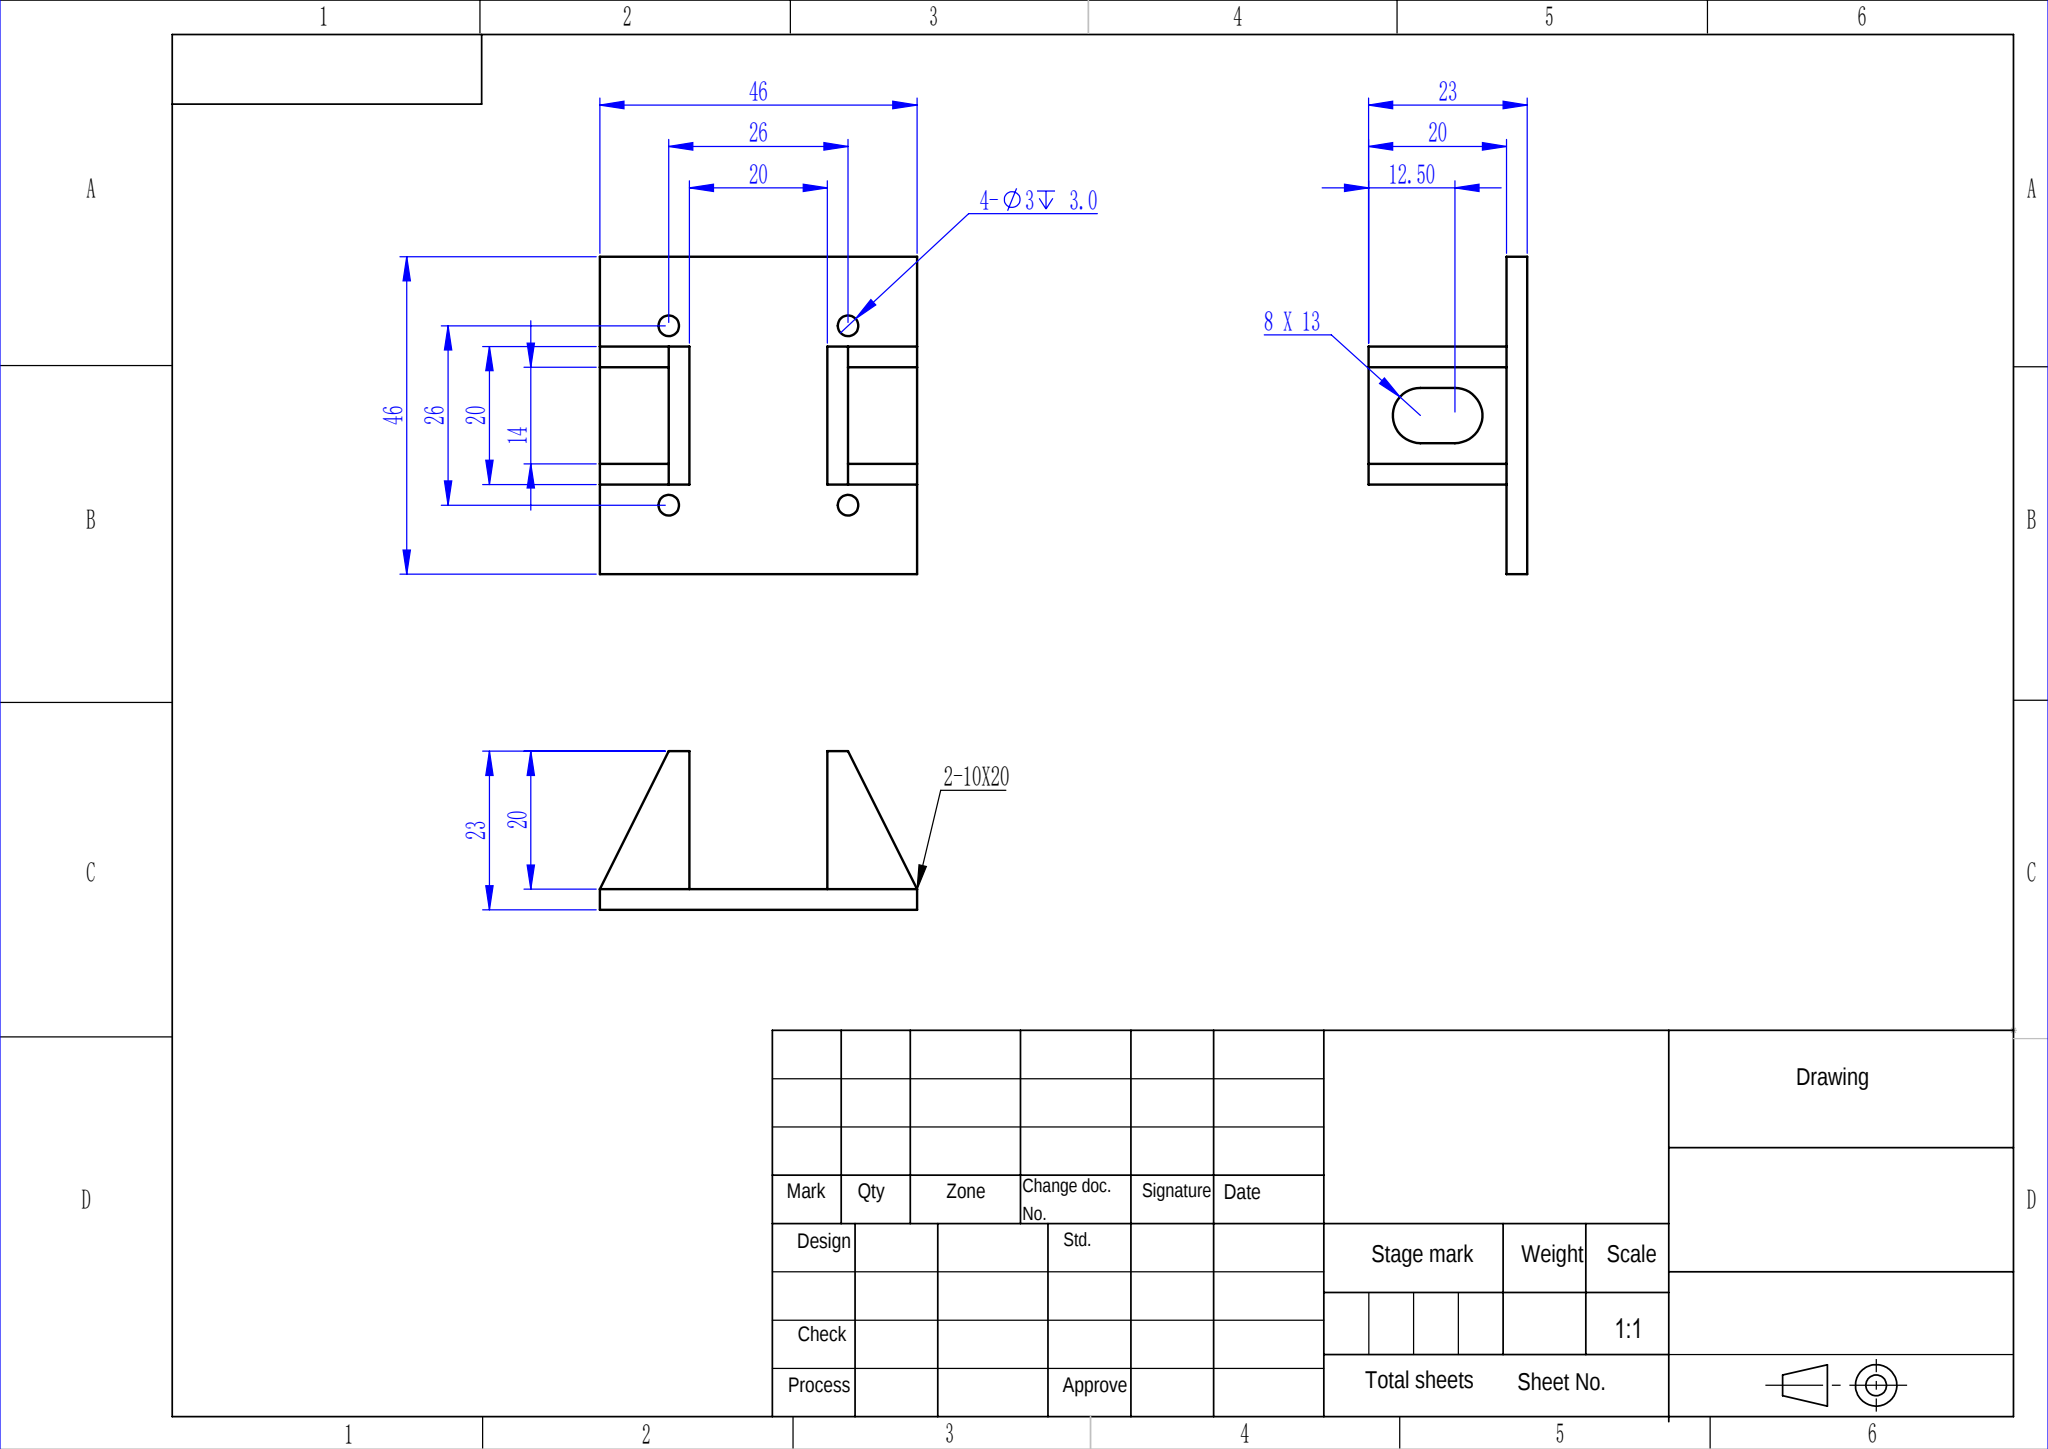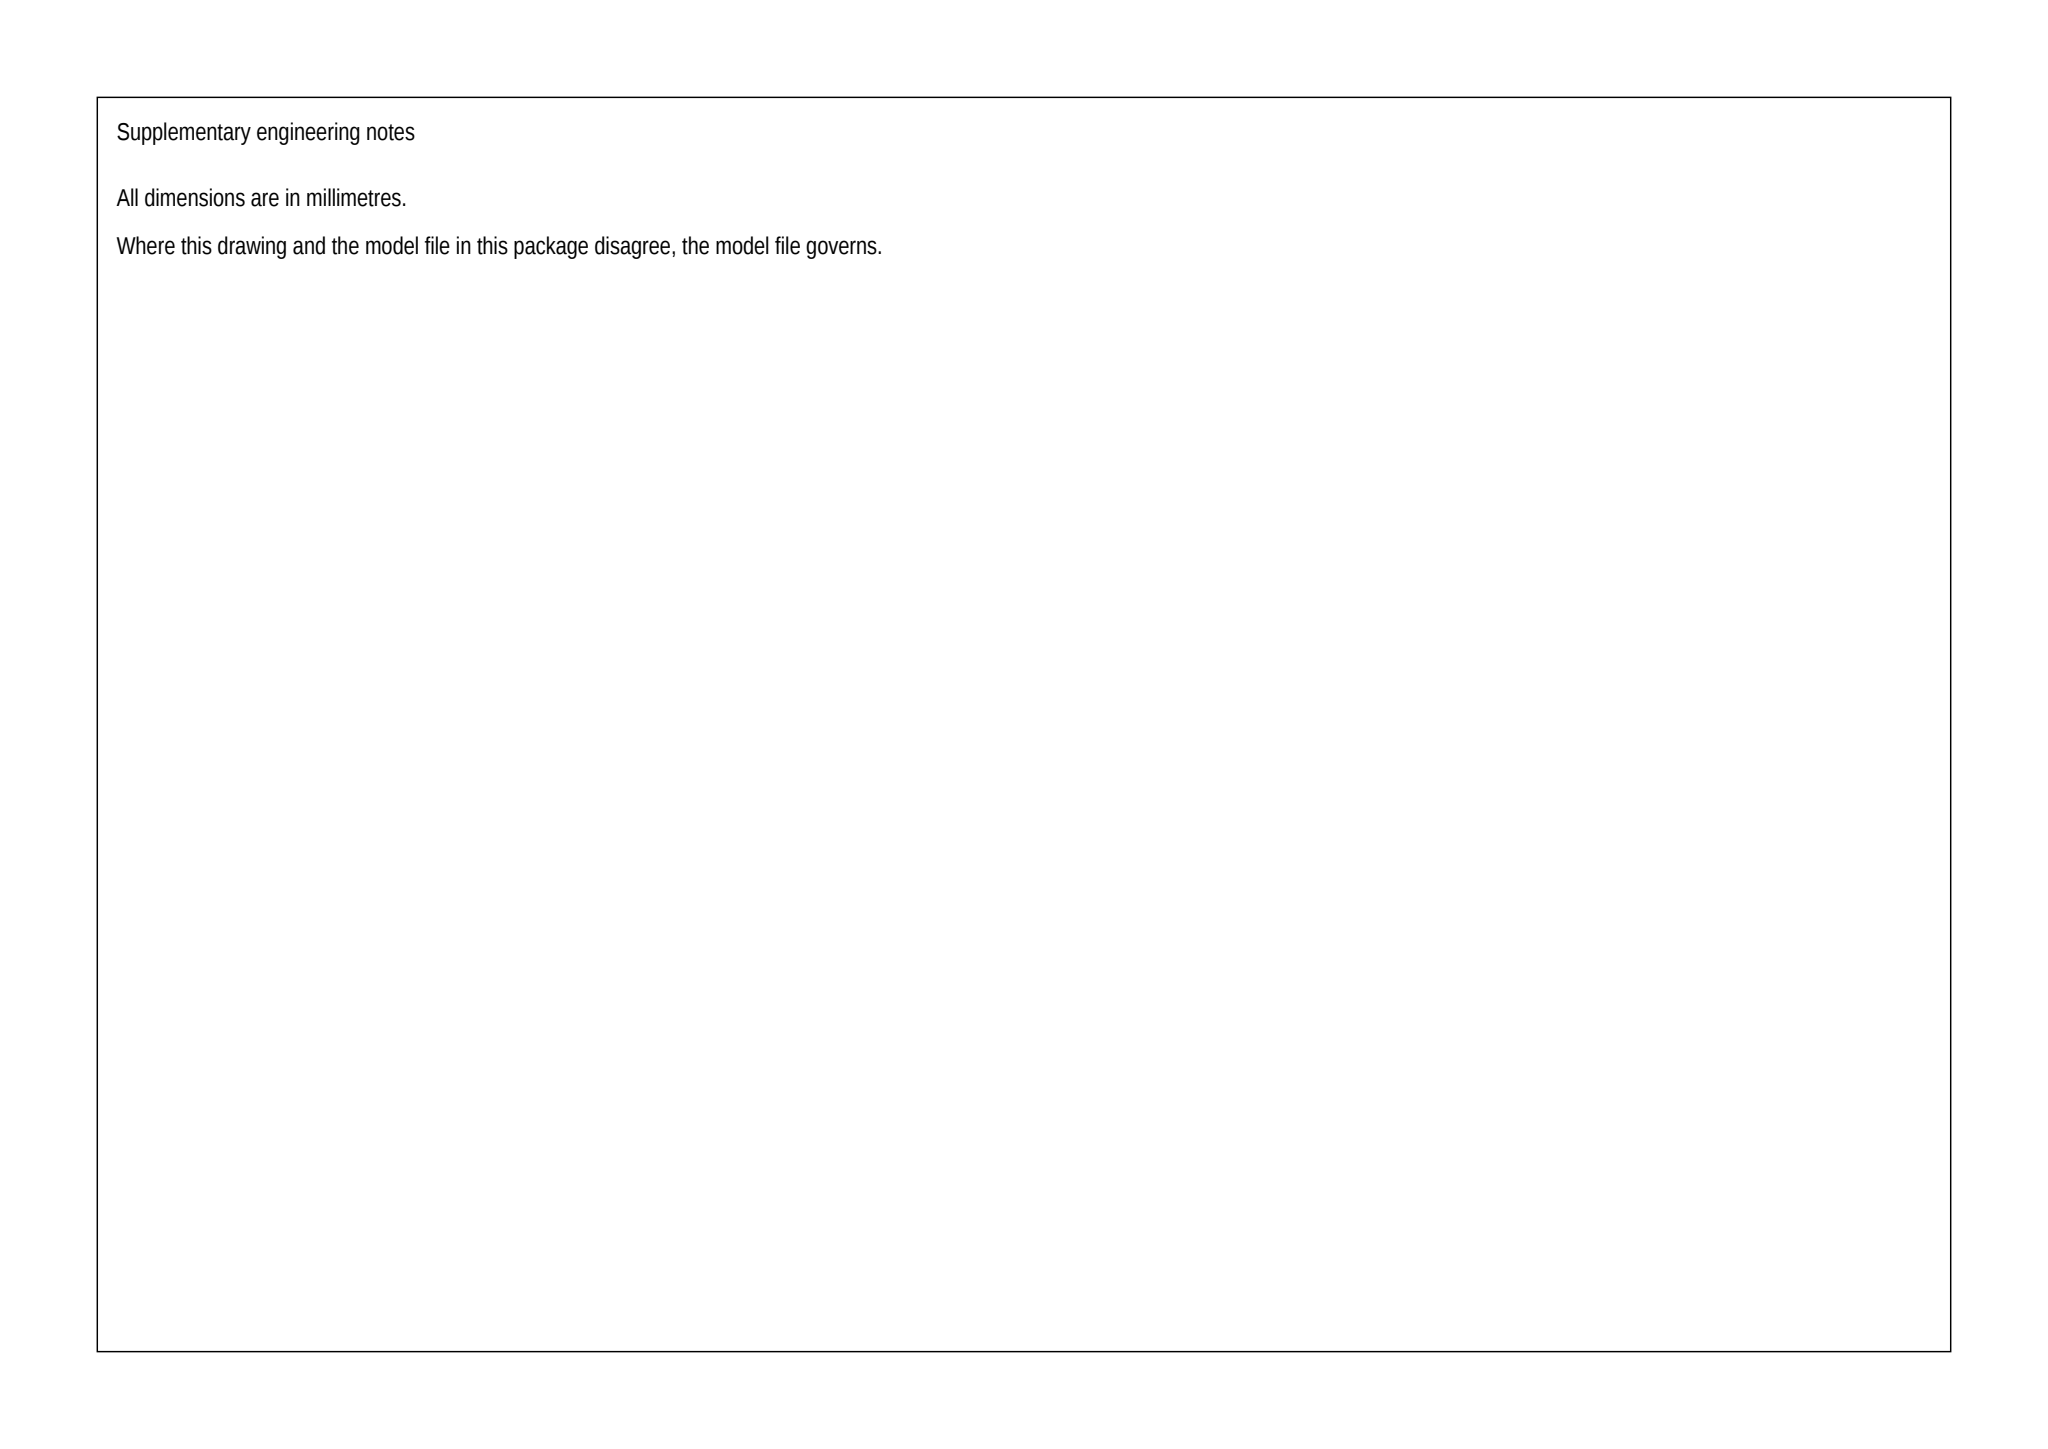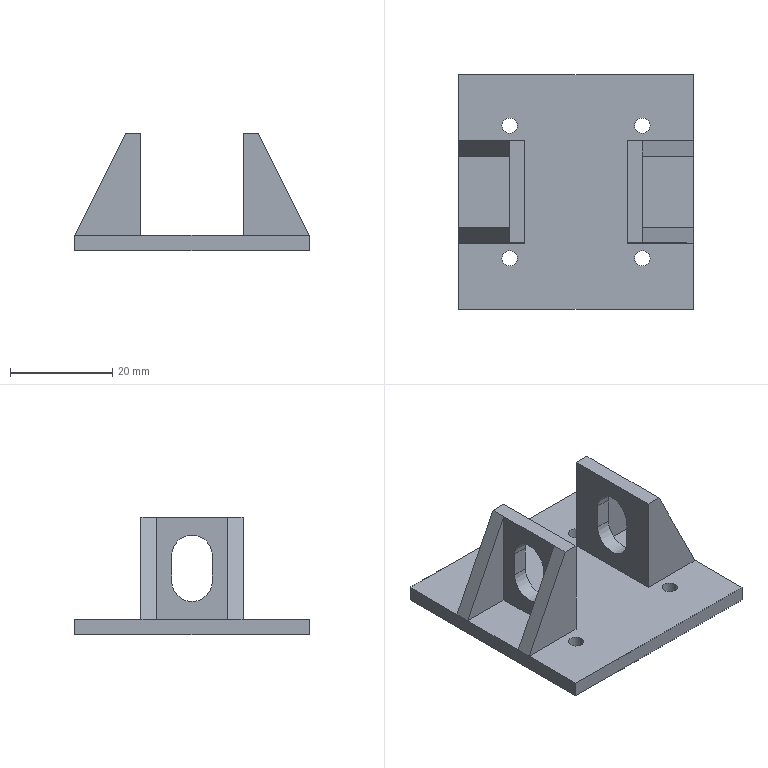Part | SolidWorks | mm | 1 solid | 42 faces | box 46 x 46 x 23 mm | volume 9322 mm3 | plane 30 | cylinder 12 | commonest cylinder face diameters 3 x8 8 x4
build123d program:
from build123d import *

# Parameters (mm, degrees)
SKETCH2_W           = 120
SKETCH2_H           = 60
BOSS_EXTRUDE1_DEPTH = 3
SKETCH3_R           = 1.5
CUT_EXTRUDE1_DEPTH  = 3
SKETCH4_R           = 1.5
CUT_EXTRUDE2_DEPTH  = 10
CUT_EXTRUDE4_DEPTH  = 57
SKETCH6_W           = 3
SKETCH6_H           = 56
BOSS_EXTRUDE3_DEPTH = 30
CUT_EXTRUDE5_REACH  = 70.425
CUT_EXTRUDE8_REACH  = 71.426
SKETCH8_W           = 48
SKETCH8_H           = 5
SKETCH8_W_2         = 5
SKETCH8_H_2         = 46
CUT_EXTRUDE9_REACH  = 66.63
SKETCH10_W          = 33
SKETCH10_H          = 5
BOSS_EXTRUDE4_DEPTH = 3
BOSS_EXTRUDE5_DEPTH = 3
CUT_EXTRUDE10_REACH = 81.63
CUT_EXTRUDE11_REACH = 78.033
CUT_EXTRUDE12_REACH = 62.614
SKETCH15_W          = 5
SKETCH15_H          = 46
SKETCH16_W          = 3
SKETCH16_H          = 20
BOSS_EXTRUDE6_DEPTH = 20
BOSS_EXTRUDE7_DEPTH = 3
BOSS_EXTRUDE8_DEPTH = 3
CUT_EXTRUDE13_DEPTH = 49.518


with BuildPart() as part:
    # Sketch2 → Boss-Extrude1 (new body)
    with BuildSketch(Plane.XY):
        Rectangle(SKETCH2_W, SKETCH2_H)
    extrude(amount=BOSS_EXTRUDE1_DEPTH)

    # Sketch3 → Cut-Extrude1 (cut)
    with BuildSketch(Plane.XY.offset(3)):
        with Locations((-41, 13)):
            Circle(SKETCH3_R)
        with Locations((-15, 13)):
            Circle(SKETCH3_R)
        with Locations((-41, -13)):
            Circle(SKETCH3_R)
        with Locations((-15, -13)):
            Circle(SKETCH3_R)
        with Locations(Location((15, -13, 0), (0, 0, 180))):
            Circle(SKETCH3_R)
        with Locations(Location((41, -13, 0), (0, 0, 180))):
            Circle(SKETCH3_R)
        with Locations(Location((15, 13, 0), (0, 0, 180))):
            Circle(SKETCH3_R)
        with Locations(Location((41, 13, 0), (0, 0, 180))):
            Circle(SKETCH3_R)
    extrude(amount=-CUT_EXTRUDE1_DEPTH, mode=Mode.SUBTRACT)

    # Sketch4 → Cut-Extrude2 (cut)
    with BuildSketch(Plane.XY.offset(3)):
        Polygon((0, -30), (0, 0), (0, 30), (-60, 30), (-60, -30), align=None)
        with Locations((-41, -13)):
            Circle(SKETCH4_R, mode=Mode.SUBTRACT)
        with Locations((-15, -13)):
            Circle(SKETCH4_R, mode=Mode.SUBTRACT)
        with Locations((-41, 13)):
            Circle(SKETCH4_R, mode=Mode.SUBTRACT)
        with Locations((-15, 13)):
            Circle(SKETCH4_R, mode=Mode.SUBTRACT)
    extrude(amount=-CUT_EXTRUDE2_DEPTH, mode=Mode.SUBTRACT)

    # Sketch5 → Cut-Extrude4 (cut)
    with BuildSketch(Plane.XY.offset(3)):
        Polygon((0, 30), (0, 28), (56, 28), (56, -28), (0, -28), (0, -30), (60, -30), (60, 30), align=None)
    extrude(amount=-CUT_EXTRUDE4_DEPTH, mode=Mode.SUBTRACT)

    # Sketch6 → Boss-Extrude3 (add)
    with BuildSketch(Plane.XY.offset(3)):
        with Locations((54.5, 0)):
            Rectangle(SKETCH6_W, SKETCH6_H)
    extrude(amount=BOSS_EXTRUDE3_DEPTH)

    # Sketch7 → Cut-Extrude5 (cut, up to next)
    with BuildSketch(Plane.ZY.offset(-53), mode=Mode.PRIVATE) as cut_extrude5_sk1:
        with BuildLine():
            Line((17, -4), (9, -4))
            ThreePointArc((9, -4), (5, 0), (9, 4))
            Line((9, 4), (17, 4))
            ThreePointArc((17, 4), (21, 0), (17, -4))
        make_face()
    cut_extrude5_tool1 = extrude(cut_extrude5_sk1.sketch, amount=-CUT_EXTRUDE5_REACH, mode=Mode.PRIVATE) & part.part
    add(cut_extrude5_tool1.solids().sort_by_distance((53, 0, 13))[0], mode=Mode.SUBTRACT)

    # Sketch8 → Cut-Extrude8 (cut, up to next)
    with BuildSketch(Plane.XY.offset(3), mode=Mode.PRIVATE) as cut_extrude8_sk1:
        with Locations((29, 25.5)):
            Rectangle(SKETCH8_W, SKETCH8_H)
    cut_extrude8_tool1 = extrude(cut_extrude8_sk1.sketch, amount=-CUT_EXTRUDE8_REACH, mode=Mode.PRIVATE) & part.part
    # Sketch8 → Cut-Extrude8 (cut, up to next)
    with BuildSketch(Plane.XY.offset(3), mode=Mode.PRIVATE) as cut_extrude8_sk2:
        with Locations((2.5, 25.5)):
            Rectangle(SKETCH8_W_2, SKETCH8_H)
    cut_extrude8_tool2 = extrude(cut_extrude8_sk2.sketch, amount=-CUT_EXTRUDE8_REACH, mode=Mode.PRIVATE) & part.part
    # Sketch8 → Cut-Extrude8 (cut, up to next)
    with BuildSketch(Plane.XY.offset(3), mode=Mode.PRIVATE) as cut_extrude8_sk3:
        with Locations((2.5, 0)):
            Rectangle(SKETCH8_W_2, SKETCH8_H_2)
    cut_extrude8_tool3 = extrude(cut_extrude8_sk3.sketch, amount=-CUT_EXTRUDE8_REACH, mode=Mode.PRIVATE) & part.part
    # Sketch8 → Cut-Extrude8 (cut, up to next)
    with BuildSketch(Plane.XY.offset(3), mode=Mode.PRIVATE) as cut_extrude8_sk4:
        with Locations((29, -25.5)):
            Rectangle(SKETCH8_W, SKETCH8_H)
    cut_extrude8_tool4 = extrude(cut_extrude8_sk4.sketch, amount=-CUT_EXTRUDE8_REACH, mode=Mode.PRIVATE) & part.part
    # Sketch8 → Cut-Extrude8 (cut, up to next)
    with BuildSketch(Plane.XY.offset(3), mode=Mode.PRIVATE) as cut_extrude8_sk5:
        with Locations((2.5, -25.5)):
            Rectangle(SKETCH8_W_2, SKETCH8_H)
    cut_extrude8_tool5 = extrude(cut_extrude8_sk5.sketch, amount=-CUT_EXTRUDE8_REACH, mode=Mode.PRIVATE) & part.part
    add(cut_extrude8_tool1.solids().sort_by_distance((29, 25.5, 3))[0], mode=Mode.SUBTRACT)
    add(cut_extrude8_tool2.solids().sort_by_distance((2.5, 25.5, 3))[0], mode=Mode.SUBTRACT)
    add(cut_extrude8_tool3.solids().sort_by_distance((2.5, 0, 3))[0], mode=Mode.SUBTRACT)
    add(cut_extrude8_tool4.solids().sort_by_distance((29, -25.5, 3))[0], mode=Mode.SUBTRACT)
    add(cut_extrude8_tool5.solids().sort_by_distance((2.5, -25.5, 3))[0], mode=Mode.SUBTRACT)

    # Sketch10 → Cut-Extrude9 (cut, up to next)
    with BuildSketch(Plane.ZY.offset(-53), mode=Mode.PRIVATE) as cut_extrude9_sk1:
        with Locations((16.5, 25.5)):
            Rectangle(SKETCH10_W, SKETCH10_H)
    cut_extrude9_tool1 = extrude(cut_extrude9_sk1.sketch, amount=-CUT_EXTRUDE9_REACH, mode=Mode.PRIVATE) & part.part
    # Sketch10 → Cut-Extrude9 (cut, up to next)
    with BuildSketch(Plane.ZY.offset(-53), mode=Mode.PRIVATE) as cut_extrude9_sk2:
        with Locations((16.5, -25.5)):
            Rectangle(SKETCH10_W, SKETCH10_H)
    cut_extrude9_tool2 = extrude(cut_extrude9_sk2.sketch, amount=-CUT_EXTRUDE9_REACH, mode=Mode.PRIVATE) & part.part
    add(cut_extrude9_tool1.solids().sort_by_distance((53, 25.5, 16.5))[0], mode=Mode.SUBTRACT)
    add(cut_extrude9_tool2.solids().sort_by_distance((53, -25.5, 16.5))[0], mode=Mode.SUBTRACT)

    # Sketch11 → Boss-Extrude4 (add)
    with BuildSketch(Plane.XZ.offset(23)):
        Polygon((53, 33), (5, 3), (53, 3), align=None)
    extrude(amount=-BOSS_EXTRUDE4_DEPTH)

    # Sketch12 → Boss-Extrude5 (add)
    with BuildSketch(Plane(origin=(0, 23, 0), x_dir=(1, 0, 0), z_dir=(0, 1, 0))):
        Polygon((53, -33), (53, -3), (5, -3), align=None)
    extrude(amount=-BOSS_EXTRUDE5_DEPTH)

    # Sketch13 → Cut-Extrude10 (cut, up to next)
    with BuildSketch(Plane(origin=(0, 23, 0), x_dir=(1, 0, 0), z_dir=(0, 1, 0)), mode=Mode.PRIVATE) as cut_extrude10_sk1:
        Polygon((56, -33), (56, -23), (37, -23), (53, -33), align=None)
    cut_extrude10_tool1 = extrude(cut_extrude10_sk1.sketch, amount=-CUT_EXTRUDE10_REACH, mode=Mode.PRIVATE) & part.part
    add(cut_extrude10_tool1.solids().sort_by_distance((49.53, 23, 26.788))[0], mode=Mode.SUBTRACT)

    # Sketch14 → Cut-Extrude11 (cut, up to next)
    with BuildSketch(Plane.XZ.offset(23), mode=Mode.PRIVATE) as cut_extrude11_sk1:
        Polygon((37, 23), (5, 3), (56, 3), (56, 23), align=None)
    cut_extrude11_tool1 = extrude(cut_extrude11_sk1.sketch, amount=-CUT_EXTRUDE11_REACH, mode=Mode.PRIVATE) & part.part
    add(cut_extrude11_tool1.solids().sort_by_distance((37.281, -23, 11.476))[0], mode=Mode.SUBTRACT)

    # Sketch15 → Cut-Extrude12 (cut, up to next)
    with BuildSketch(Plane.XY.offset(3), mode=Mode.PRIVATE) as cut_extrude12_sk1:
        with Locations((53.5, 0)):
            Rectangle(SKETCH15_W, SKETCH15_H)
    cut_extrude12_tool1 = extrude(cut_extrude12_sk1.sketch, amount=-CUT_EXTRUDE12_REACH, mode=Mode.PRIVATE) & part.part
    add(cut_extrude12_tool1.solids().sort_by_distance((53.5, 0, 3))[0], mode=Mode.SUBTRACT)

    # Sketch16 → Boss-Extrude6 (add)
    with BuildSketch(Plane.XY.offset(3)):
        with Locations((16.5, 0)):
            Rectangle(SKETCH16_W, SKETCH16_H)
        with Locations((39.5, 0)):
            Rectangle(SKETCH16_W, SKETCH16_H)
    extrude(amount=BOSS_EXTRUDE6_DEPTH)

    # Sketch17 → Boss-Extrude7 (add)
    with BuildSketch(Plane.XZ.offset(10)):
        Polygon((5, 3), (15, 3), (15, 23), align=None)
        Polygon((41, 23), (41, 3), (51, 3), align=None)
    extrude(amount=-BOSS_EXTRUDE7_DEPTH)

    # Sketch18 → Boss-Extrude8 (add)
    with BuildSketch(Plane(origin=(0, 10, 0), x_dir=(1, 0, 0), z_dir=(0, 1, 0))):
        Polygon((51, -3), (41, -3), (41, -23), align=None)
        Polygon((15, -23), (15, -3), (5, -3), align=None)
    extrude(amount=-BOSS_EXTRUDE8_DEPTH)

    # Sketch19 → Cut-Extrude13 (cut, through all)
    with BuildSketch(Plane.ZY.offset(-15)):
        with BuildLine():
            Line((10.5, 4), (15.5, 4))
            ThreePointArc((15.5, 4), (19.5, 0), (15.5, -4))
            Line((15.5, -4), (10.5, -4))
            ThreePointArc((10.5, -4), (6.5, 0), (10.5, 4))
        make_face()
    extrude(amount=-CUT_EXTRUDE13_DEPTH, mode=Mode.SUBTRACT)


solid = part.part